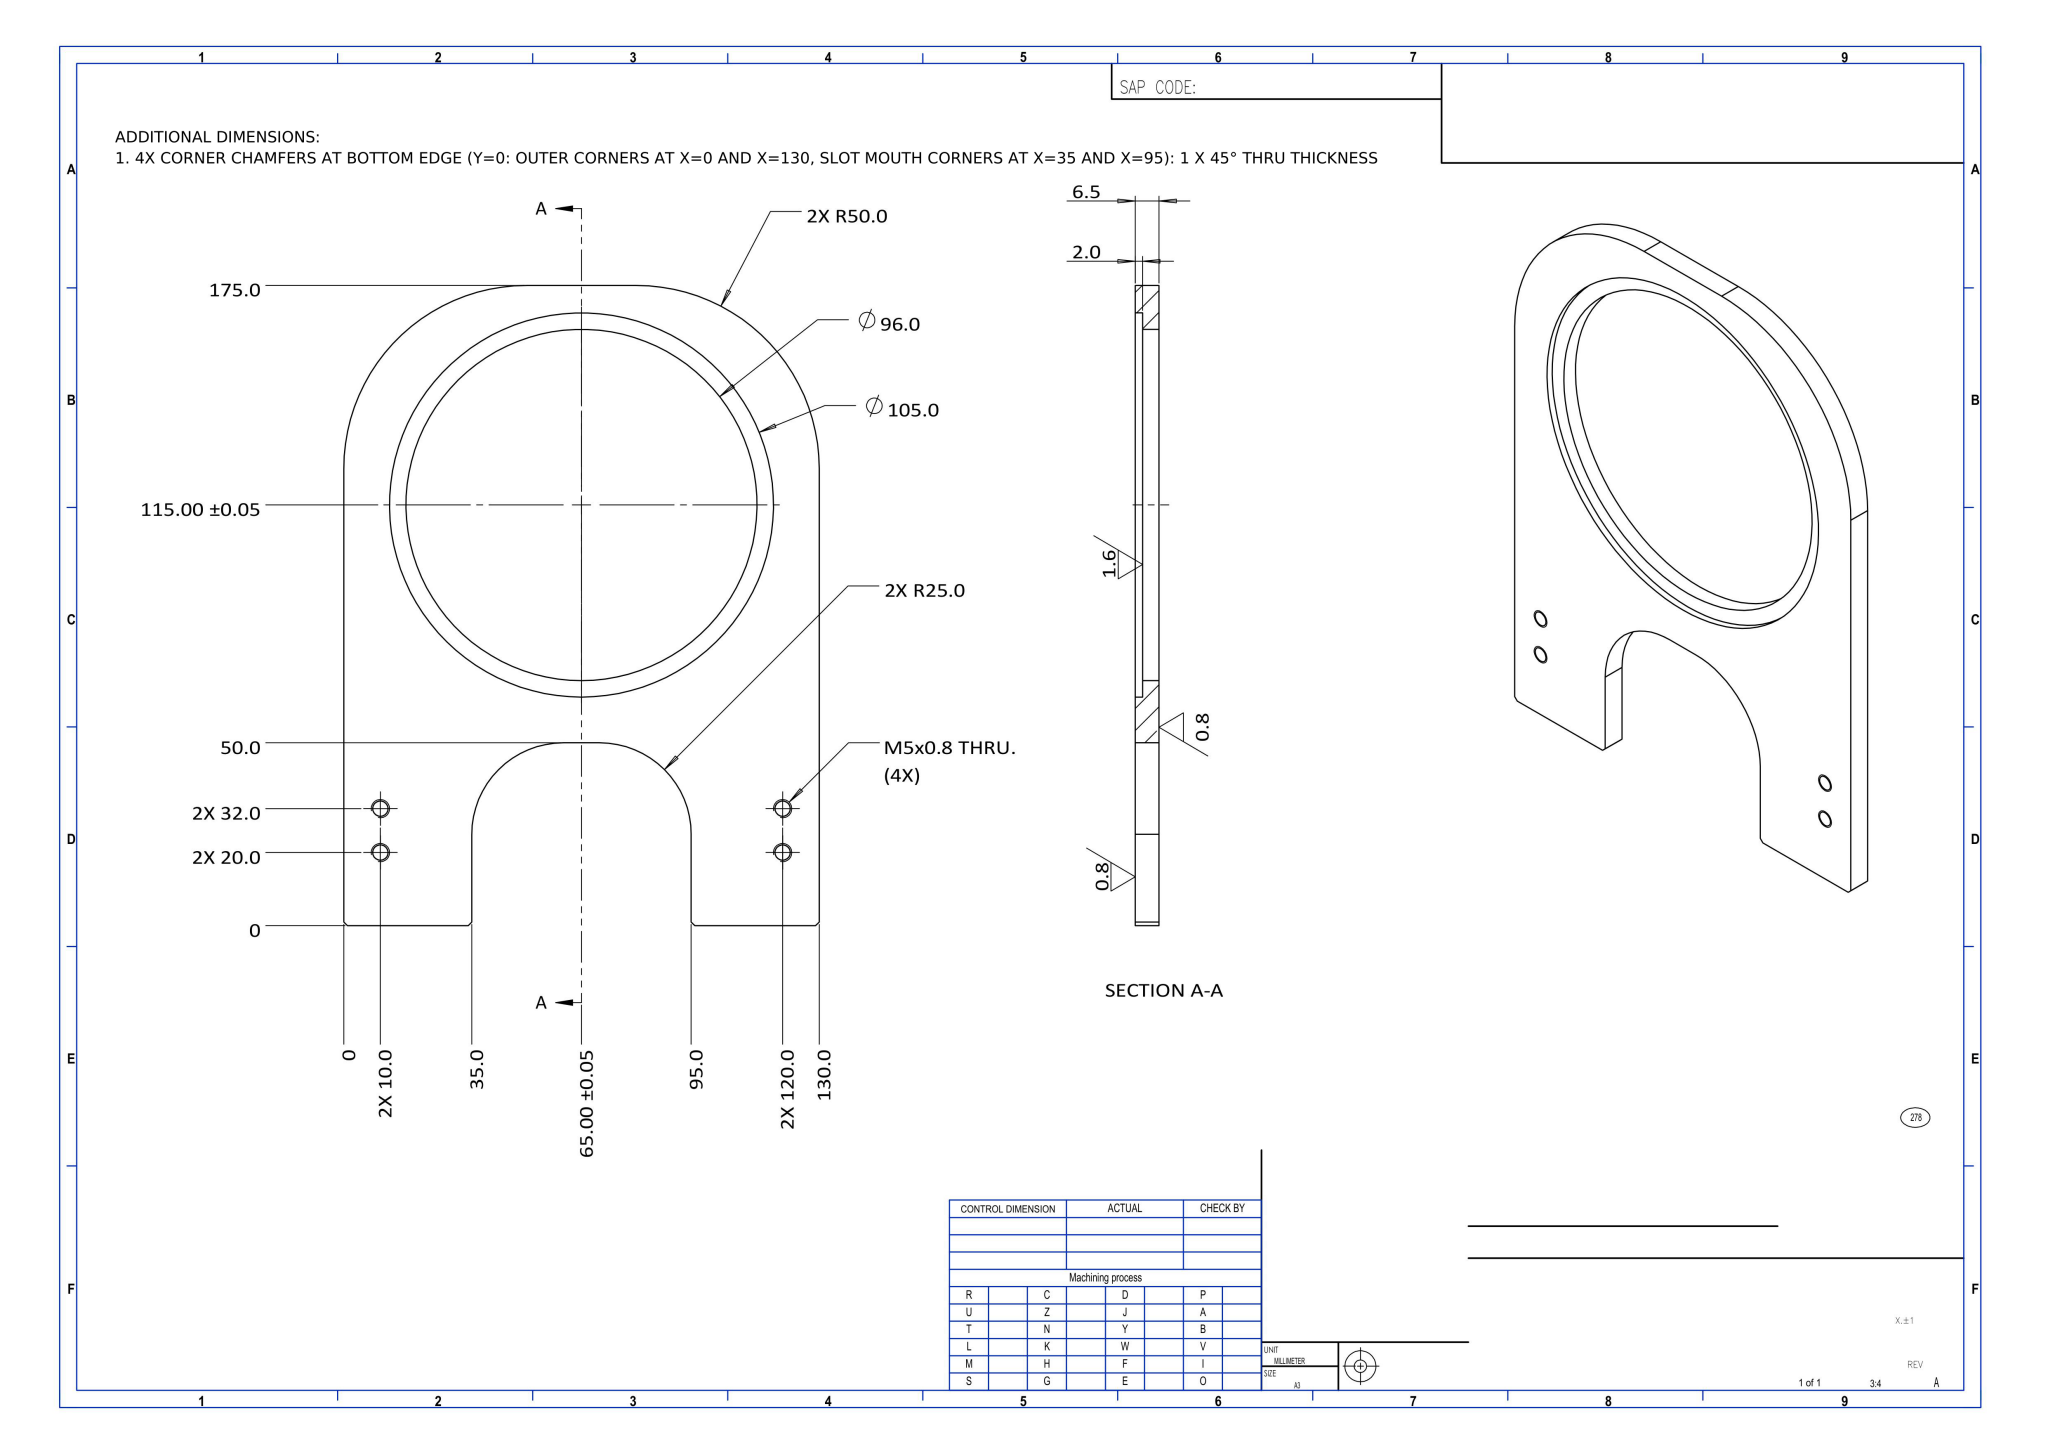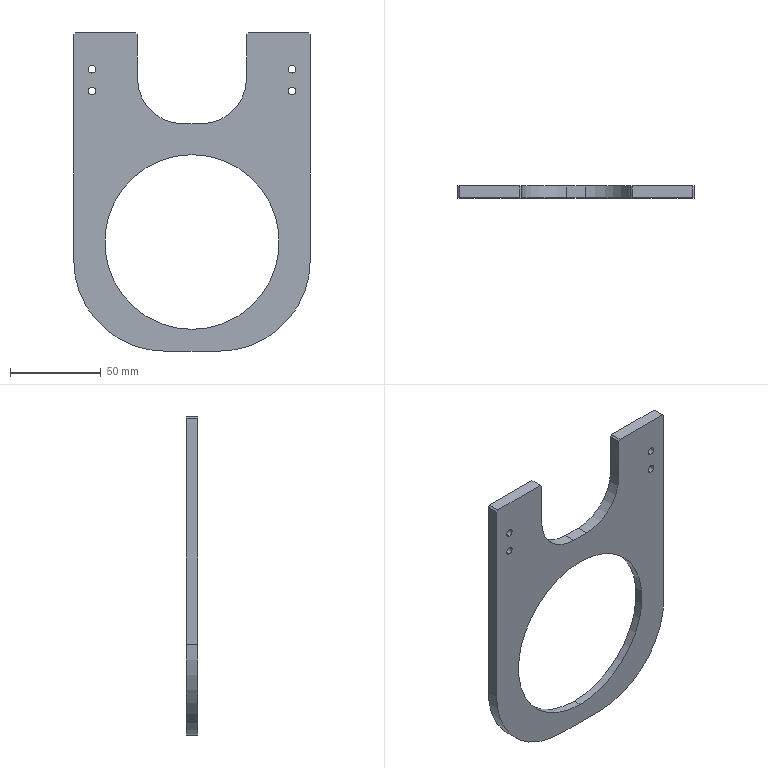Part | NX | mm | 1 solid | 31 faces | box 130 x 6.5 x 175 mm | volume 72881 mm3 | cylinder 16 | plane 15 | commonest cylinder face diameters 4.2 x8 105 x2 96 x2 100 x2 50 x2